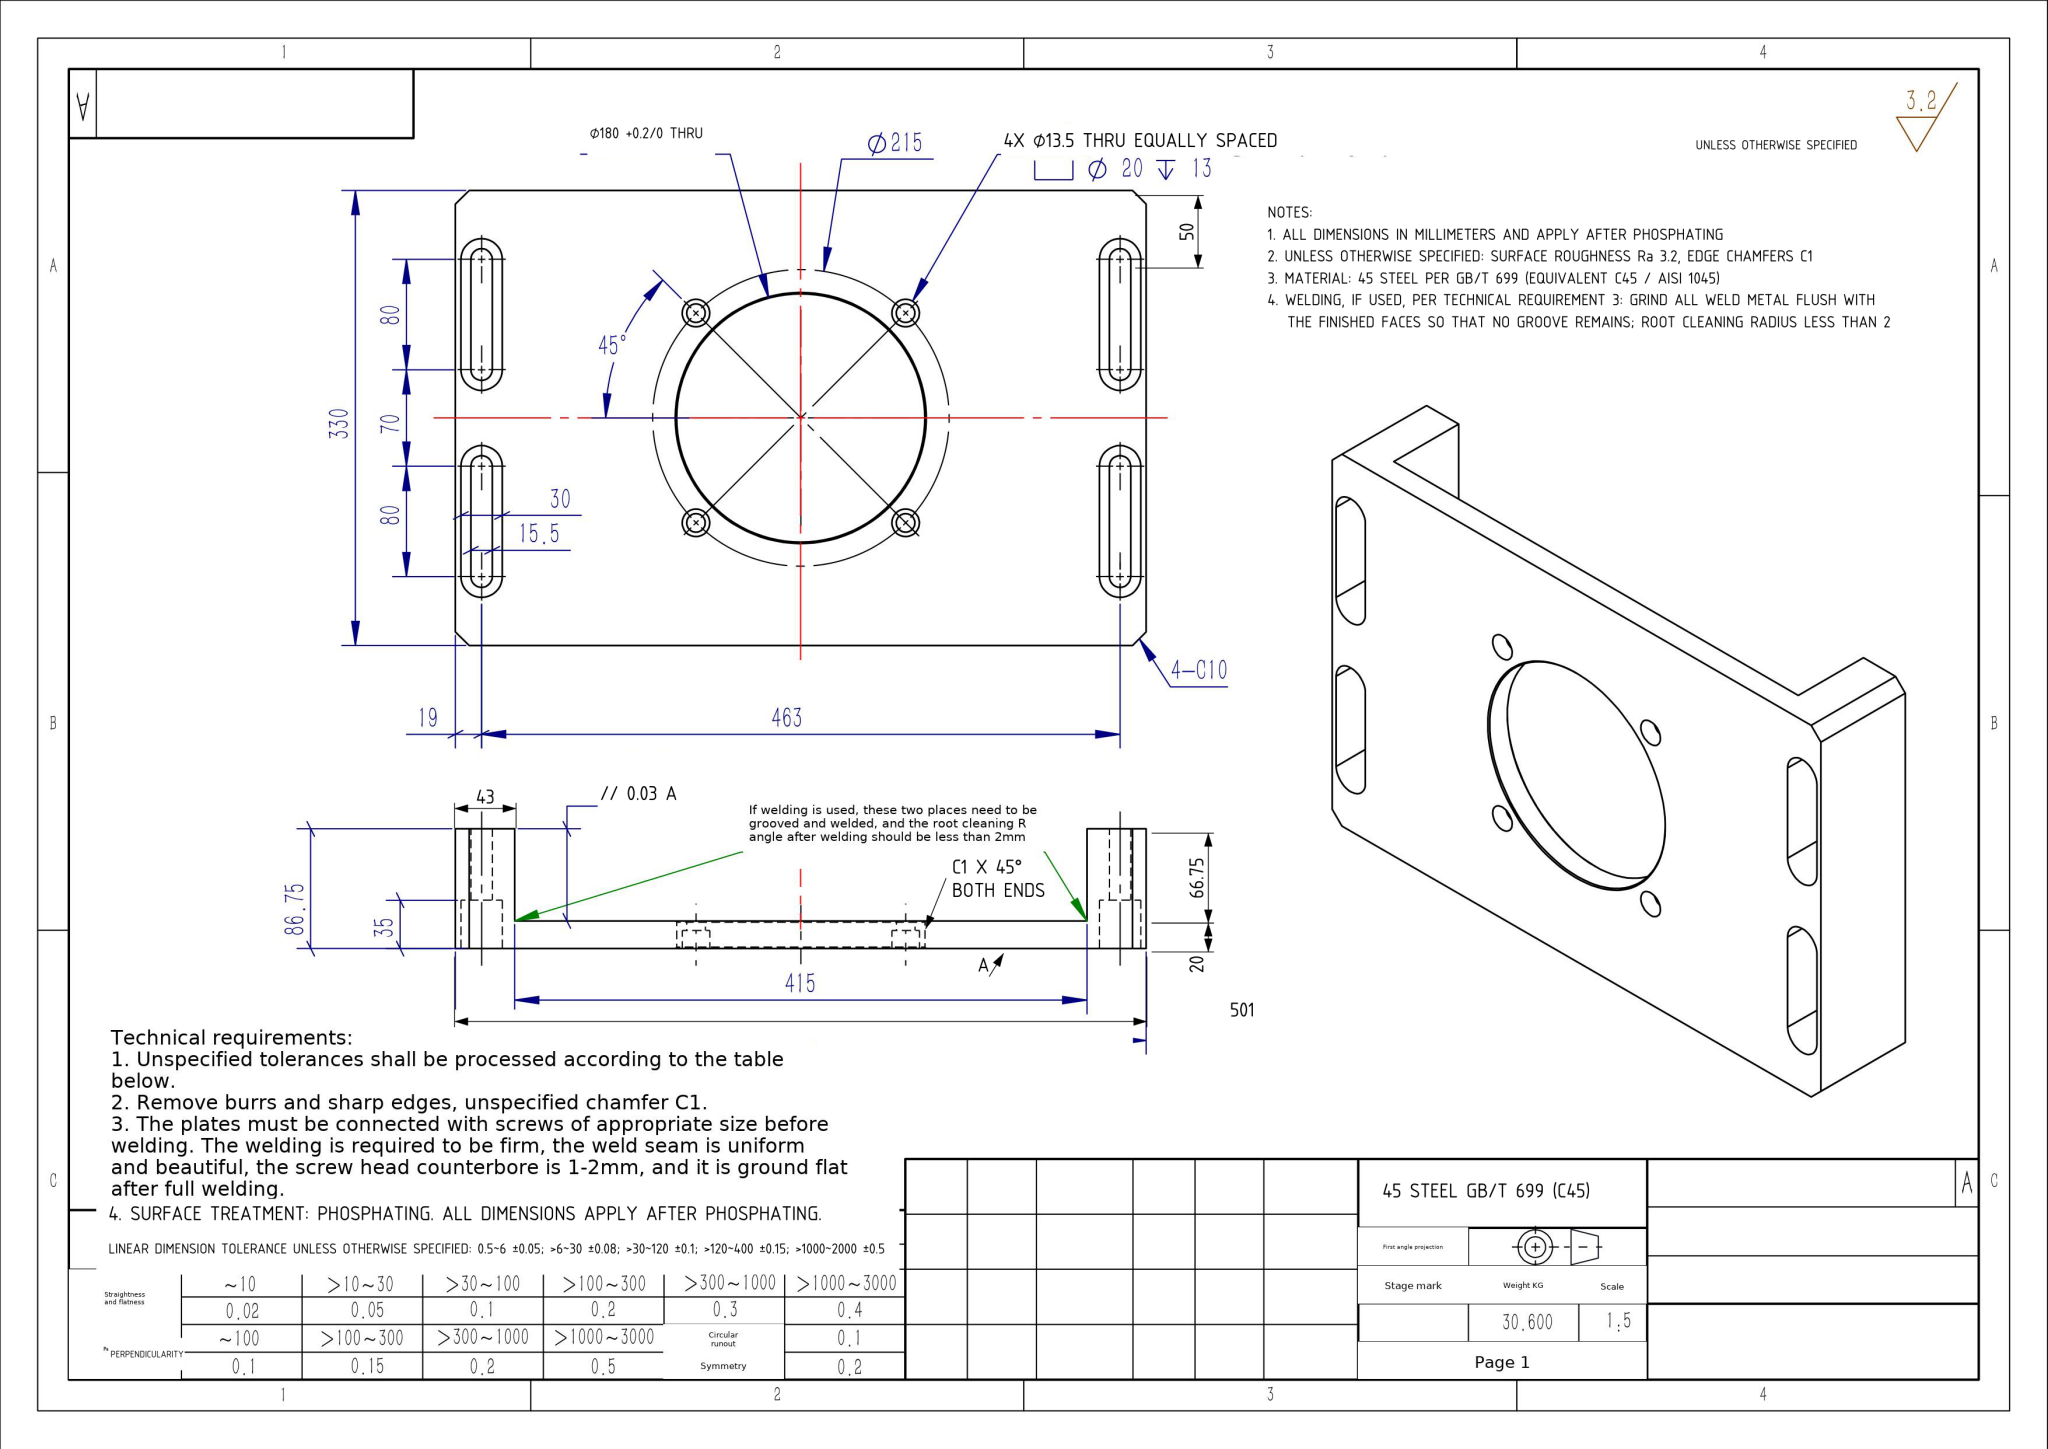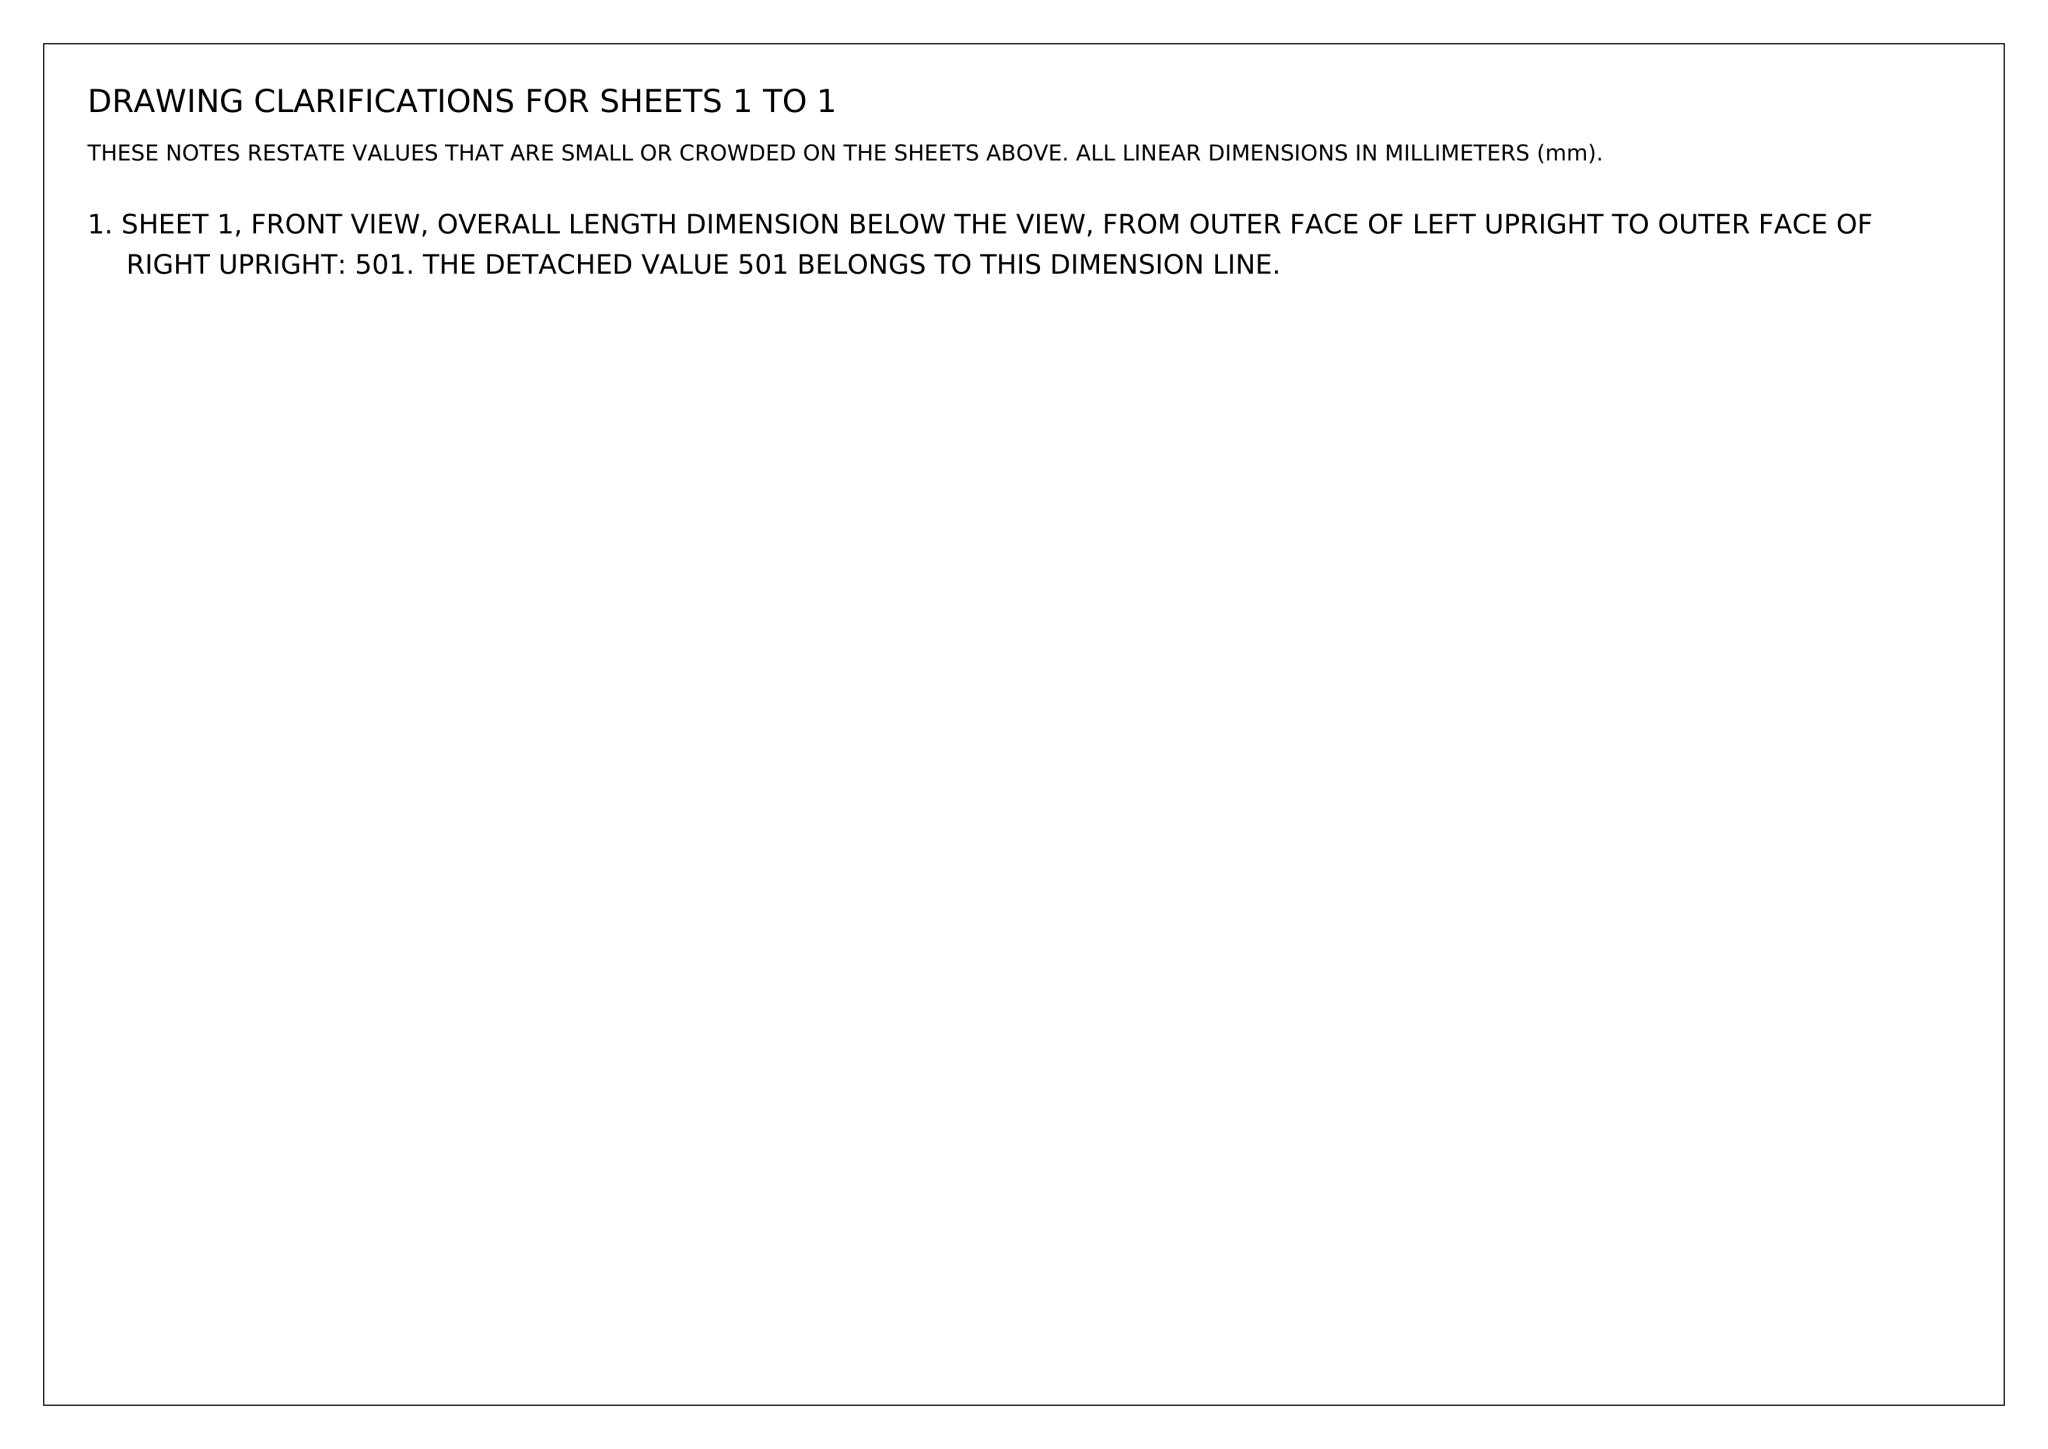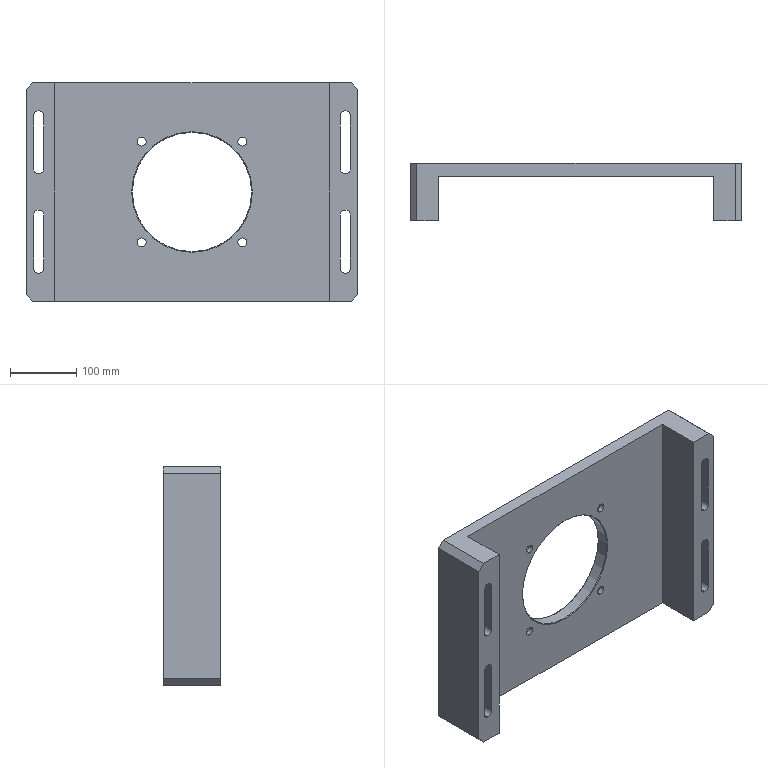Part | NX | mm | 1 solid | 80 faces | box 501 x 86.75 x 330 mm | volume 3923066 mm3 | cylinder 38 | plane 38 | cone 4 | commonest cylinder face diameters 15.5 x12 20 x8 13.5 x8 30 x8 180 x2